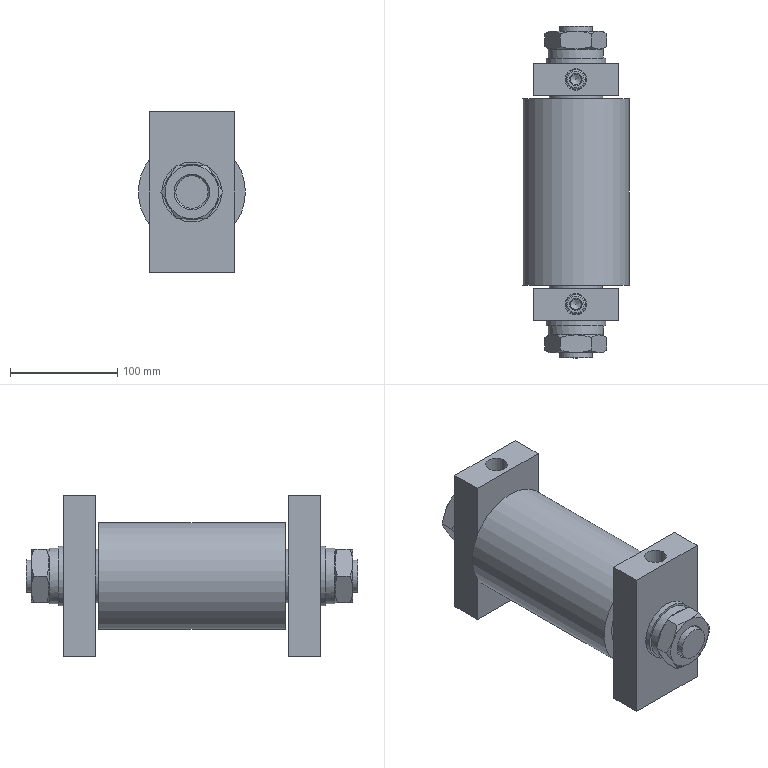Assembly | NX | mm | 16 component files | 46 solids | 255 faces | box 100 x 310 x 150 mm | volume 1849035 mm3 | plane 106 | cylinder 59 | cone 54 | sphere 28 | torus 8 | commonest cylinder face diameters 13.5 x6 50 x5 59.014 x4 2.5 x4 30.158 x4 80 x4 60.001 x4 45.8 x2
Bill of materials:
GB-T848-2002,M33 | 2 |  | Flat annular ring (washer-like): a thin disc with a concentric circular through-hole, flat parallel faces, and plain cylindrical inner and outer edges.
GB93-87,(33) | 2 |  | Single Coil Spring Lock Washer, Normal Type, GB 93-87,(33)
GB-T292_AC-1994,7010_AC | 2 |  | Annular assembly that looks like a radial ball bearing: concentric outer and inner rings with a single row of spherical rolling elements in the radial gap between them. No cage or shields are visible.
GB-T70.1-2000,M12x90 | 2 |  | Hexagon Socket Head Cap Screw, GB-T 70.1-2000,M12x90
unnamed part 1 | 2 |  | Rectangular block with one large round through-bore across its largest face, plus a smaller round hole running down from the narrow top face that crosses the large bore.
unnamed part 2 | 1 |  | Stepped round shaft, symmetric end to end. It has a long large-diameter middle section, a step down to a medium diameter at each end, and a smaller end section beyond that. Each medium-diameter step has a radial cross-hole, and there are narrow grooves near both ends of the middle section.
GB-T6172_1-2000,M33x3.5 | 2 |  | Hexagon Thin Nut, Chamfered, GB-T 6172.1-2000,M33x3.5
unnamed part 3 | 2 |  | Thin, flat, open ring (split circular band) with two tabs at the gap, each tab having a small round hole. The band looks wider at the top, opposite the gap, and narrower toward the tabs.
unnamed part 4 | 1 |  | Plain cylindrical tube or sleeve with a straight concentric through-bore and flat, square-cut ends.
Mates:
1. fix | Shaft 1 component
2. concentric | Bearing 2 edge | Shaft 1 edge
3. concentric | Bearing 1 edge | Shaft 1 edge
4. concentric | Snap_ring 2 edge | Shaft 1 edge
5. concentric | Snap_ring 1 edge | Shaft 1 edge
6. concentric | Idler 1 edge | Bearing 2 edge
7. touch align | Bracket 2 face | Shaft 1 face
8. distance | Bracket 2 face | Idler 1 face
9. concentric | GB-T848-2002_M33 2 edge | Bracket 2 edge
10. concentric | GB93-87__33 2 edge | GB-T848-2002_M33 2 edge
11. concentric | GB-T6172_1-2000_M33x3_5 2 edge | GB93-87__33 2 edge
12. touch align | Bracket 1 face | Shaft 1 face
13. distance | Bracket 1 face | Idler 1 face
14. concentric | Set_screw 1 edge | Bracket 1 edge
15. concentric | GB-T848-2002_M33 1 edge | Bracket 1 edge
16. concentric | GB93-87__33 1 edge | GB-T848-2002_M33 1 edge
17. concentric | GB-T6172_1-2000_M33x3_5 1 edge | GB93-87__33 1 edge